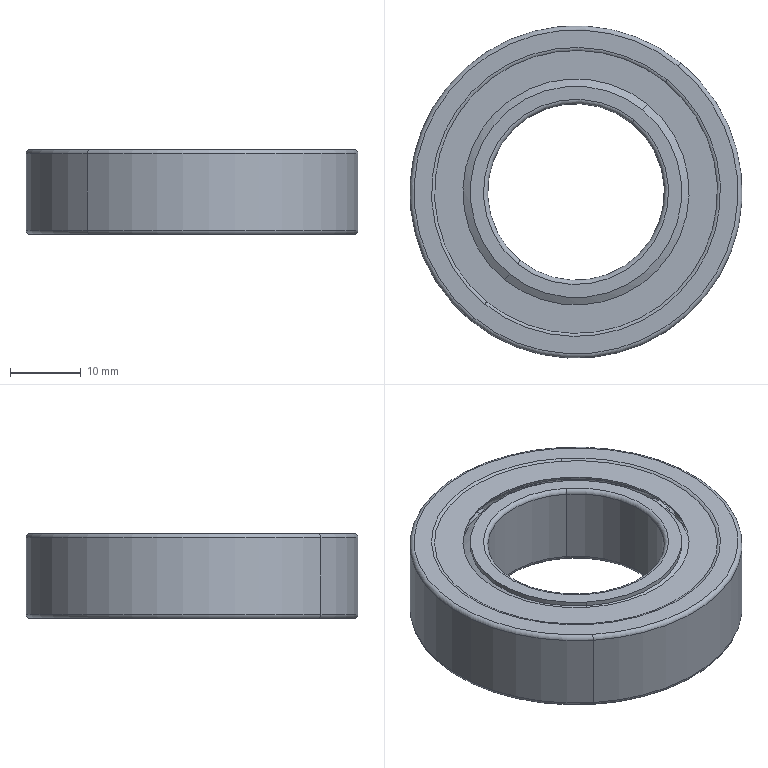Component | SolidWorks | 12AEncoderWheel-1_12A6005RZBearing-1 | 33 solids | 428 faces | volume 10631 mm3 | sphere 192 | cylinder 110 | plane 100 | torus 22 | cone 4 | commonest cylinder face diameters 37.1 x47 34.9 x47 39.667 x4 29.889 x4 32.333 x4 47 x2 25 x2